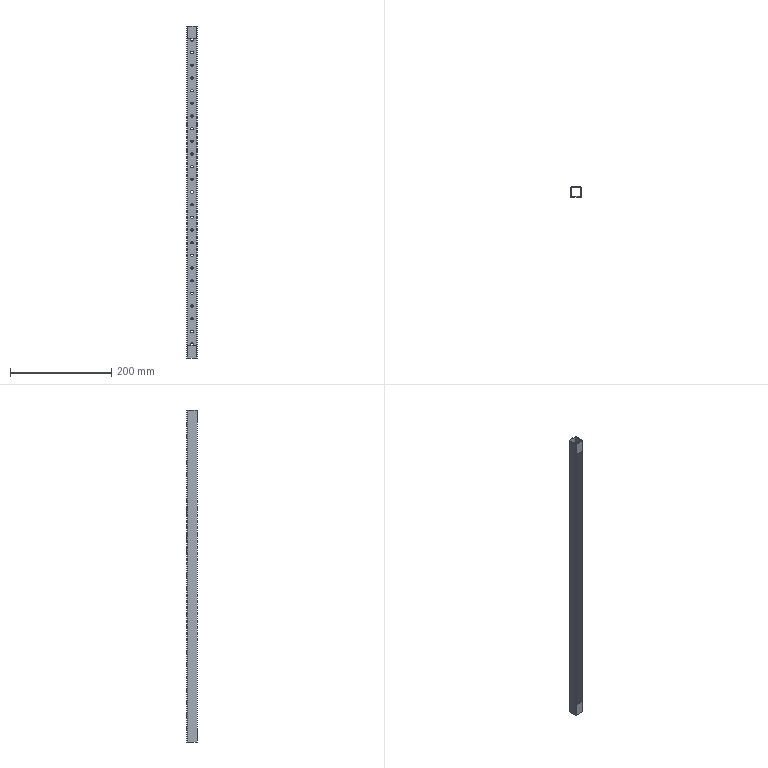Component | SolidWorks | FrontDoorAssembly-1_FrontDoorWelding-1_FrontDoorTransverseStiffenerPG50-02-103-1 | 3 solids | 80 faces | volume 55773 mm3 | cylinder 48 | plane 26 | cone 6 | commonest cylinder face diameters 4.6 x40 5 x4 3.3 x2 0.3 x2 | material AISI 1045 Steel, cold drawn